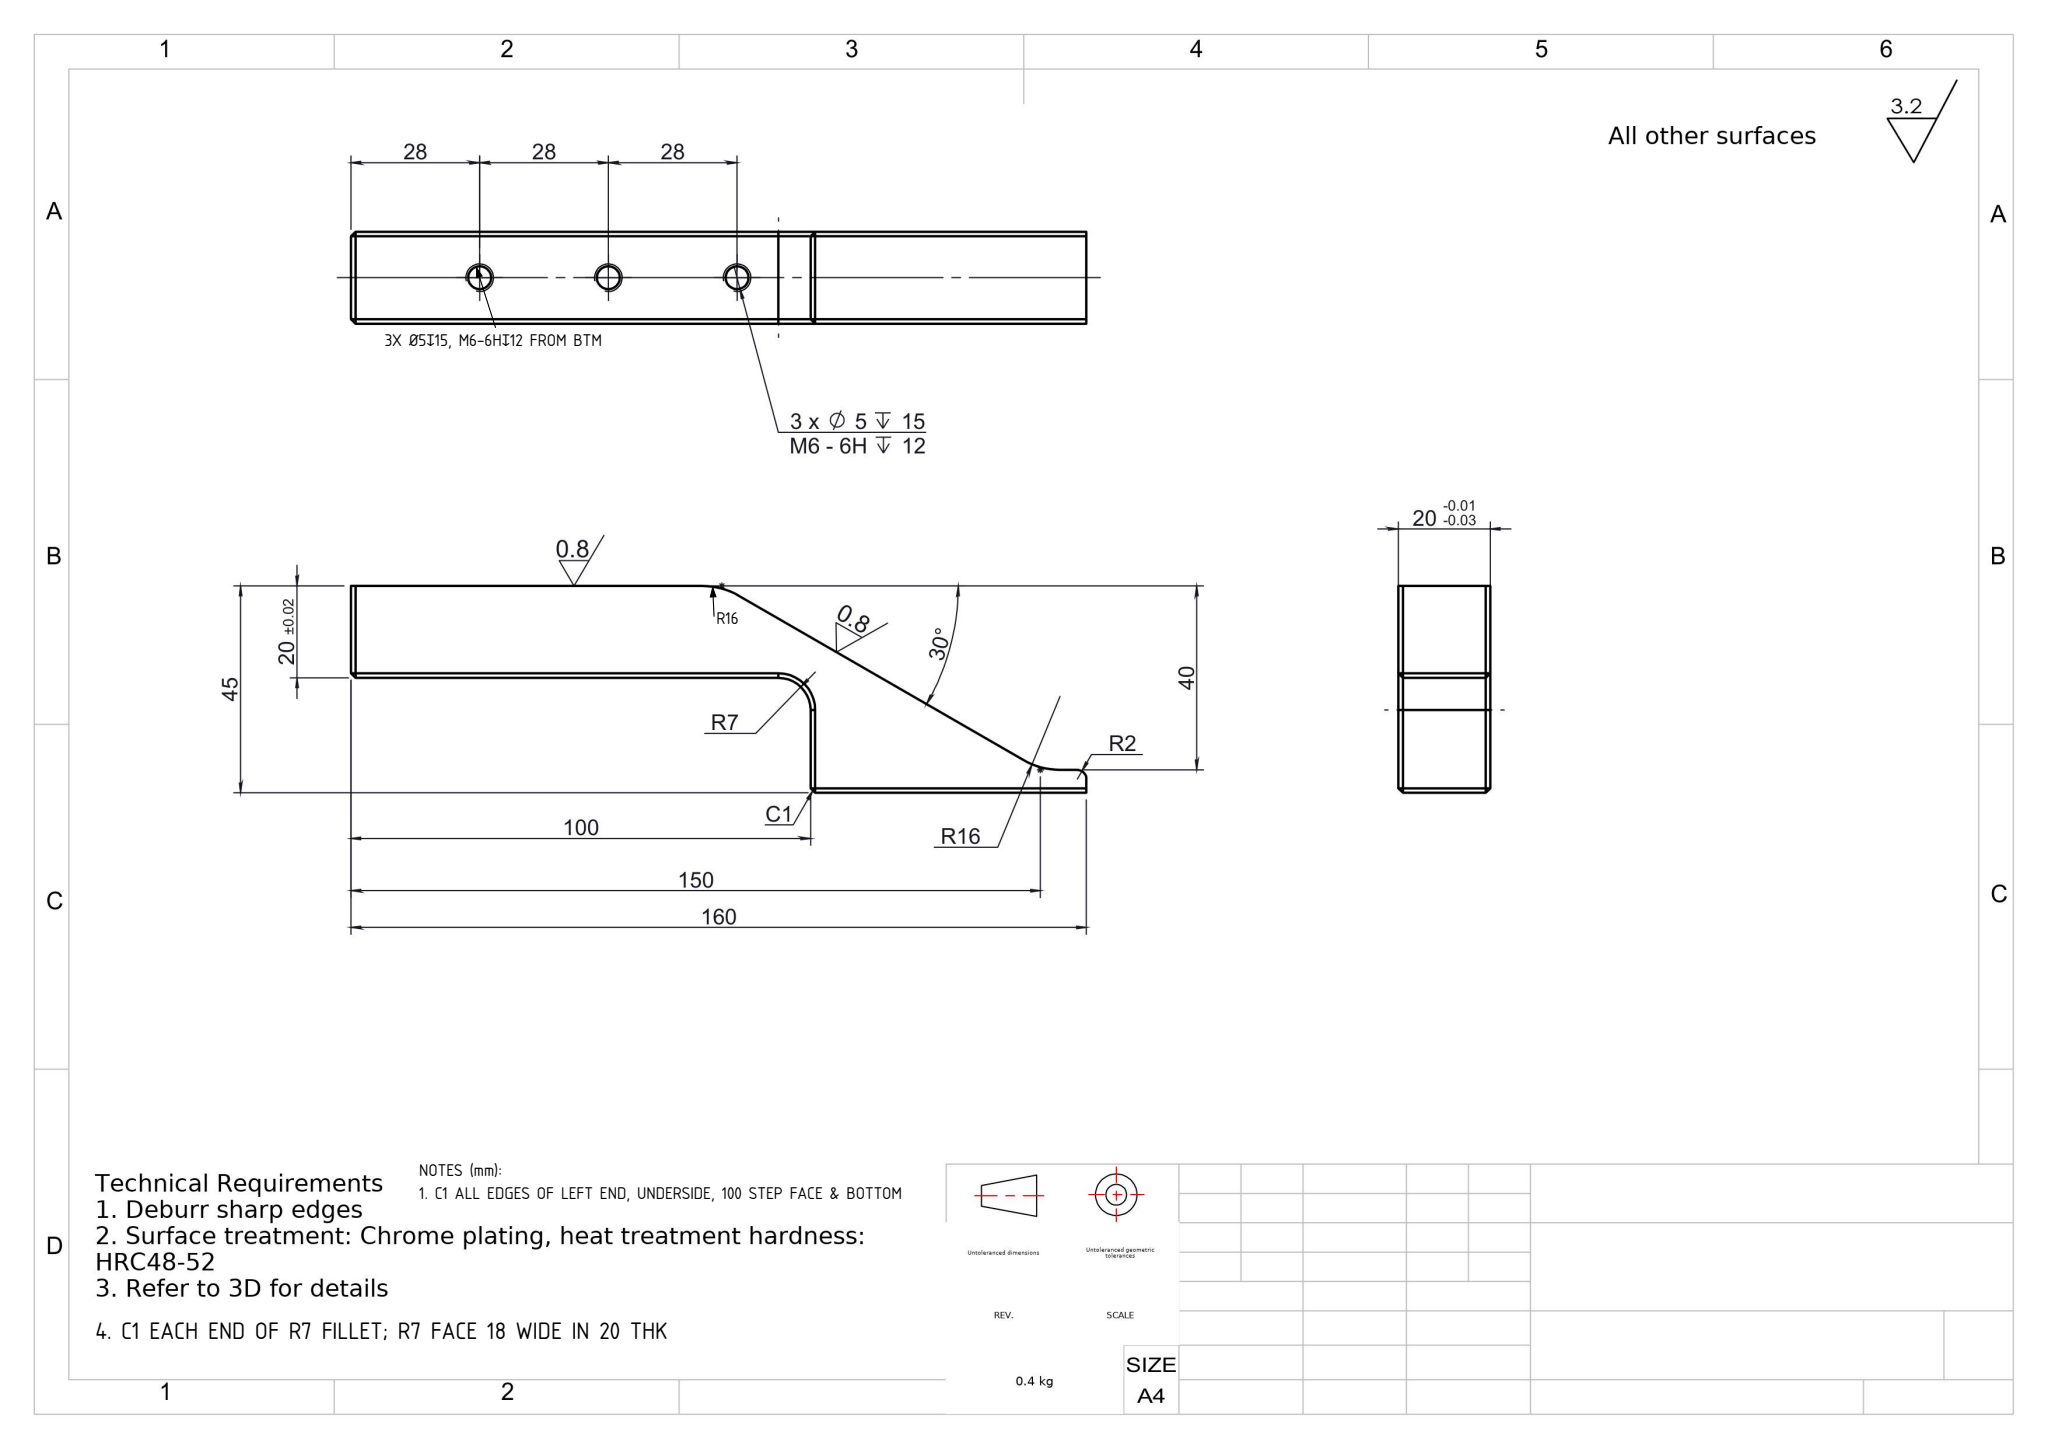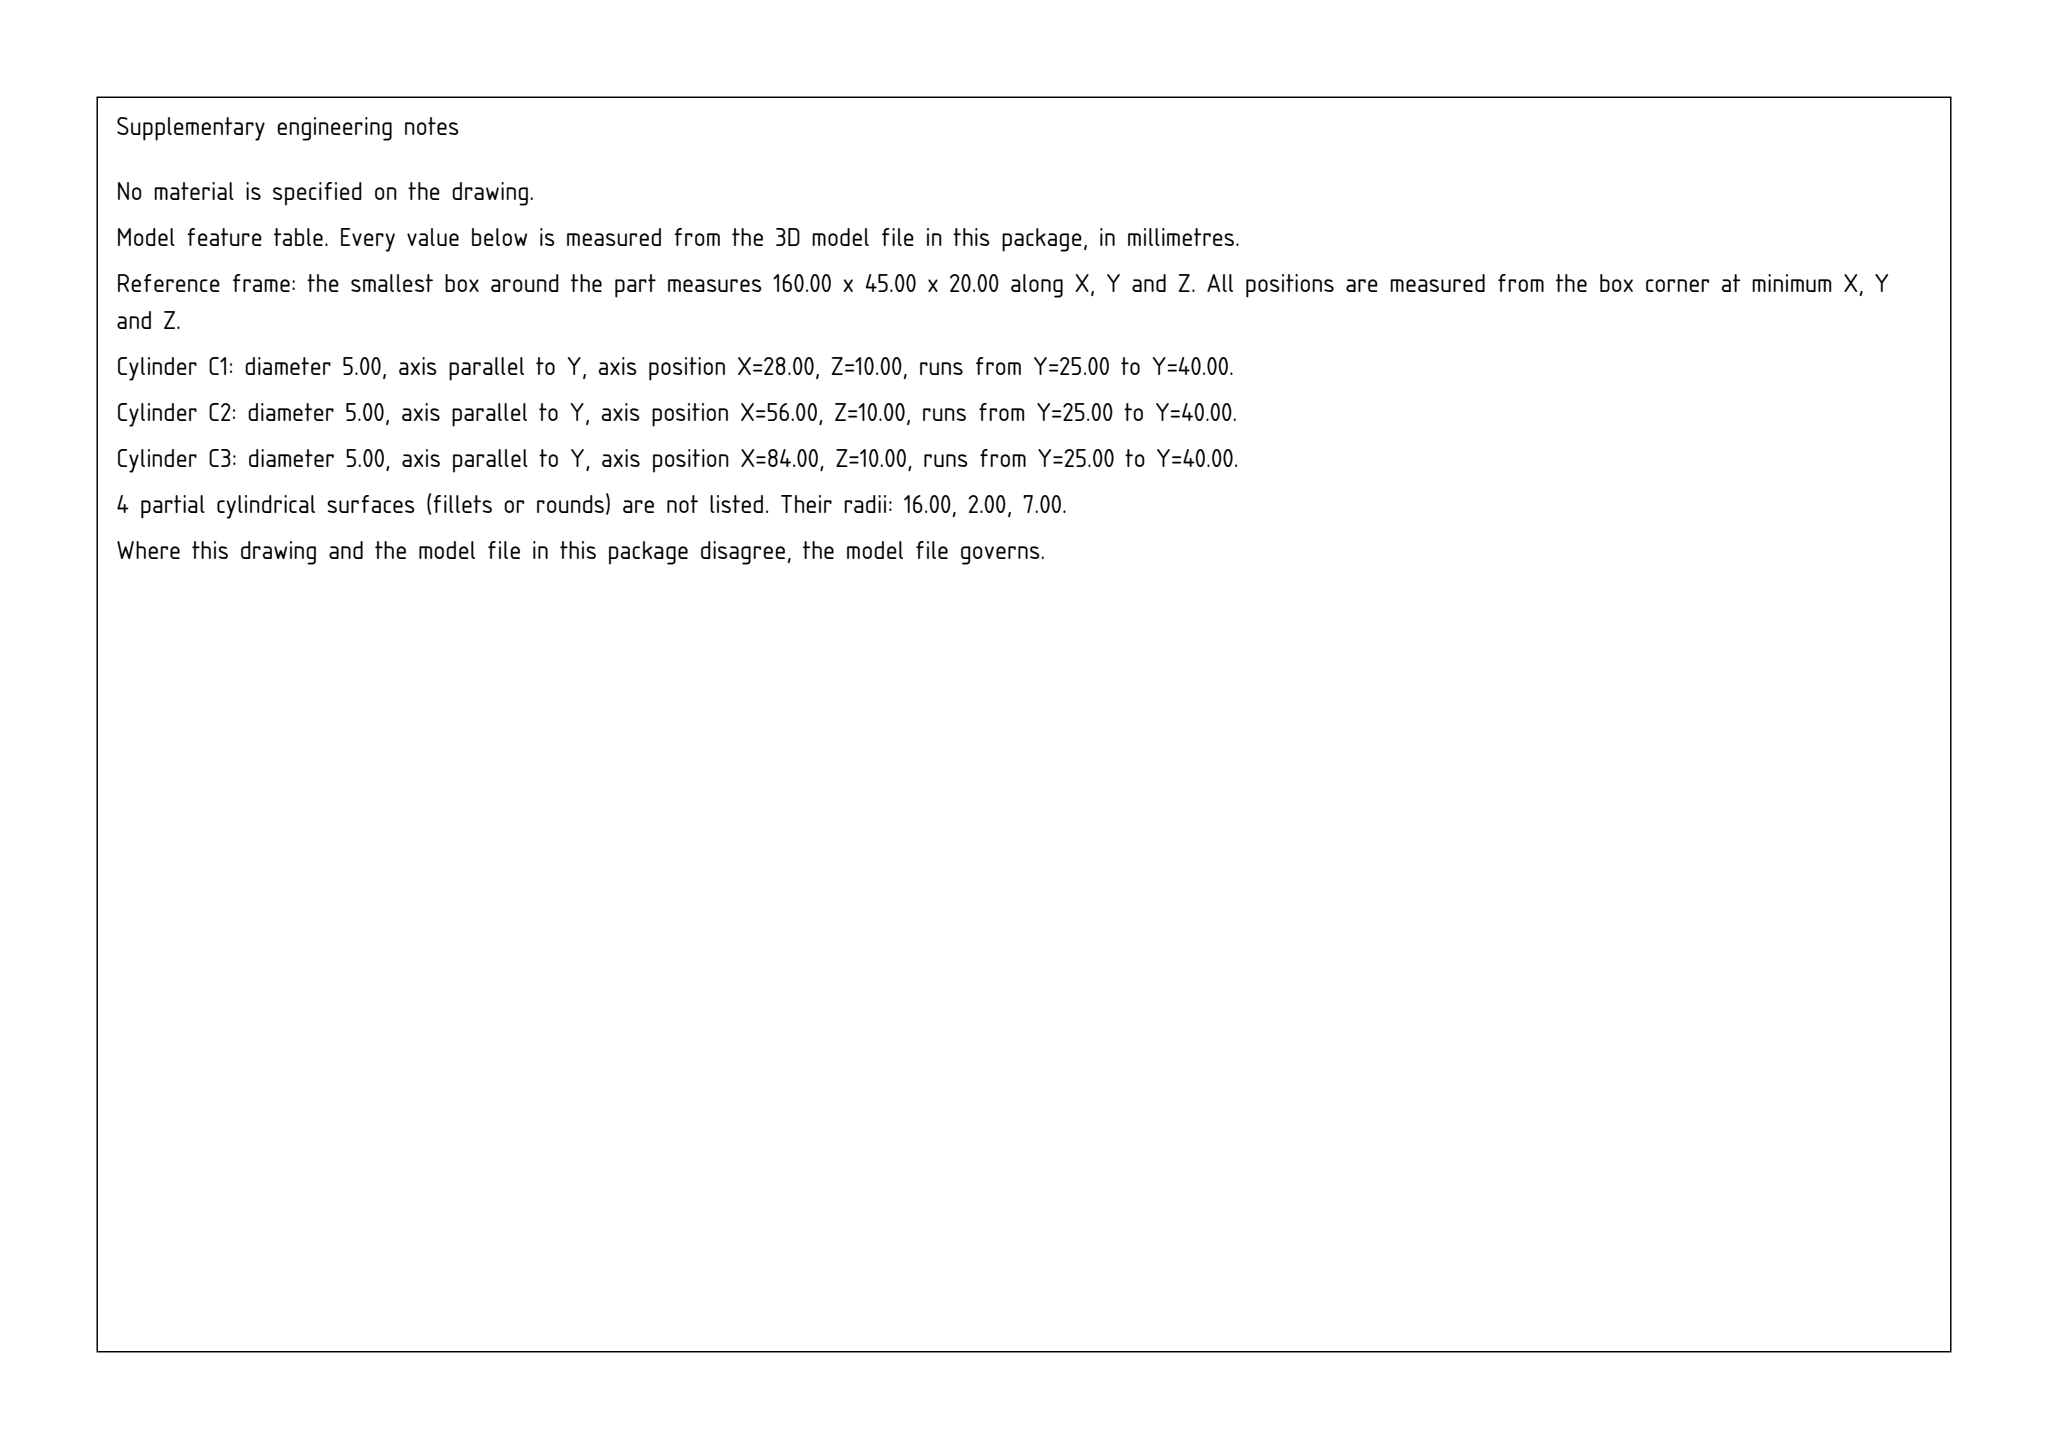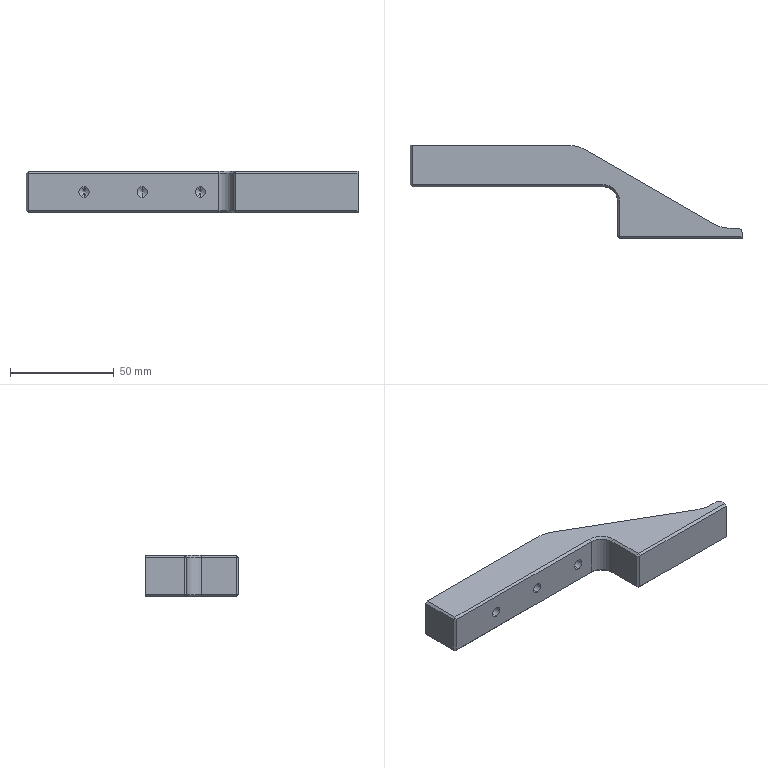Part | SolidWorks | mm | material Cr12 | 1 solid | 42 faces | box 160 x 45 x 20 mm | volume 57347 mm3 | plane 24 | cylinder 10 | cone 8 | commonest cylinder face diameters 5 x6 32 x2 14 x1 4 x1
Drawing notes:
R16 BLEND TOP FACE TO 30 DEG SLOPE, CTR 76.43 FROM LH END, 29 UP | from the solid: cylinder dia 32 (R16), axis z, center (76.43, 29), len 20 - tangent to top face y=45
C1 EACH END OF R7 FILLET; R7 FACE 18 WIDE IN 20 THK | from the solid: cylinder dia 14 (R7) at (93,18), length 18 in 20 thk; cones 90 deg incl, ref dia 16, qty 2
3X Ø5 DP 15, M6-6H DP 12 DRILLED UP FROM UNDERSIDE OF 20 THK ARM | from the solid: Ø5 holes, axis y, at x=28/56/84, z=10, from y=25 to y=40, 118° point cones at y=40
C1 ALL EDGES OF LEFT END, UNDERSIDE, 100 STEP FACE & BOTTOM | from the solid: 45° planes 1x1 at x=0, y=25 (x1-93), x=100, y=0 (x101-160) plus 54.7° corner facets
build123d program:
from build123d import *

# Parameters (mm, degrees)
SKETCH1_W             = 150
SKETCH1_H             = 45
BOSS_EXTRUDE1_DEPTH   = 10
CUT_EXTRUDE1_DEPTH    = 81.816
FILLET1_R             = 16
SKETCH4_W             = 100
SKETCH4_H             = 25
CUT_EXTRUDE2_DEPTH    = 81.816
SKETCH5_W             = 20
SKETCH5_H             = 5
BOSS_EXTRUDE2_DEPTH   = 10
FILLET2_R             = 16
FILLET3_R             = 7
M6_TAPPED_HOLE1_D     = 5
M6_TAPPED_HOLE1_DEPTH = 15
M6_TAPPED_HOLE1_TIP   = 1.502
CHAMFER1_SIZE         = 1
FILLET4_R             = 2


with BuildPart() as part:
    # Sketch1 → Boss-Extrude1 (new, symmetric)
    with BuildSketch(Plane.XY):
        Rectangle(SKETCH1_W, SKETCH1_H)
    extrude(amount=BOSS_EXTRUDE1_DEPTH, both=True)

    # Sketch2 → Cut-Extrude1 (cut, through all)
    with BuildSketch(Plane.XY.offset(10)):
        Polygon((5.718, 22.5), (75, 22.5), (75, -17.5), align=None)
    extrude(amount=-CUT_EXTRUDE1_DEPTH, mode=Mode.SUBTRACT)

    # Fillet1
    fillet1_edges = [part.edges().sort_by_distance(p)[0] for p in [
        (5.718, 22.5, 0),
    ]]
    fillet(fillet1_edges, radius=FILLET1_R)

    # Sketch4 → Cut-Extrude2 (cut, through all)
    with BuildSketch(Plane.XY.offset(10)):
        with Locations((-25, -10)):
            Rectangle(SKETCH4_W, SKETCH4_H)
    extrude(amount=-CUT_EXTRUDE2_DEPTH, mode=Mode.SUBTRACT)

    # Sketch5 → Boss-Extrude2 (add)
    with BuildSketch(Plane(origin=(75, 0, 0), x_dir=(0, 0, -1), z_dir=(1, 0, 0))):
        with Locations((0, -20)):
            Rectangle(SKETCH5_W, SKETCH5_H)
    extrude(amount=BOSS_EXTRUDE2_DEPTH)

    # Fillet2
    fillet2_edges = [part.edges().sort_by_distance(p)[0] for p in [
        (75, -17.5, 0),
    ]]
    fillet(fillet2_edges, radius=FILLET2_R)

    # Fillet3
    fillet3_edges = [part.edges().sort_by_distance(p)[0] for p in [
        (25, 2.5, 0),
    ]]
    fillet(fillet3_edges, radius=FILLET3_R)

    # M6 Tapped Hole1
    with Locations(Plane(origin=(0, 2.5, 0), x_dir=(-1, 0, 0), z_dir=(0, -1, 0))):
        with Locations((47, 0), (19, 0), (-9, 0)):
            Hole(M6_TAPPED_HOLE1_D / 2, depth=M6_TAPPED_HOLE1_DEPTH)
            with Locations((0, 0, -(M6_TAPPED_HOLE1_DEPTH + M6_TAPPED_HOLE1_TIP / 2))):  # 118° drill point
                Cone(0, M6_TAPPED_HOLE1_D / 2, M6_TAPPED_HOLE1_TIP, mode=Mode.SUBTRACT)

    # Chamfer1
    chamfer1_edges = [part.edges().sort_by_distance(p)[0] for p in [
        (-75, 12.5, 10),
        (55, -22.5, -10),
        (55, -22.5, 10),
        (-75, 2.5, 0),
        (25, -13.5, -10),
        (25, -22.5, 0),
        (25, -13.5, 10),
        (-75, 12.5, -10),
        (-28.5, 2.5, 10),
        (-28.5, 2.5, -10),
        (22.95, 0.4497, 10),
        (22.95, 0.4497, -10),
    ]]
    chamfer(chamfer1_edges, length=CHAMFER1_SIZE)

    # Fillet4
    fillet4_edges = [part.edges().sort_by_distance(p)[0] for p in [
        (85, -17.5, 0),
    ]]
    fillet(fillet4_edges, radius=FILLET4_R)


solid = part.part